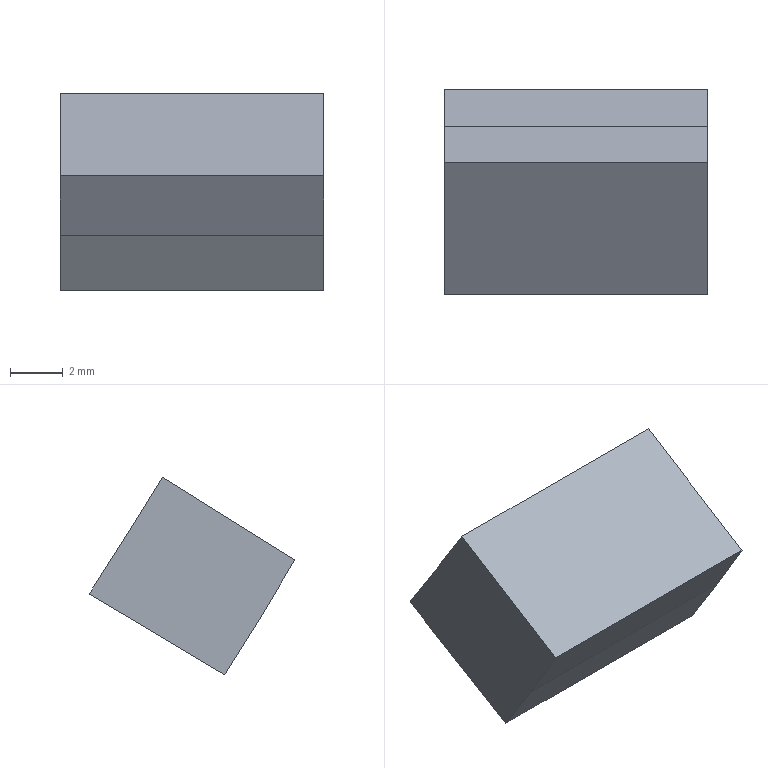Component | SolidWorks | Key5x5x16-2 | 1 solid | 8 faces | box 10 x 7.8 x 7.49 mm | volume 308 mm3 | plane 8
build123d program:
from build123d import *

# Parameters (mm, degrees)
BOSS_EXTRUDE1_DEPTH = 10


with BuildPart() as part:
    # Sketch1 → Boss-Extrude1 (new body)
    with BuildSketch(Plane.XY):
        Polygon((5.447, 152.957), (2.855, 152.957), (2.855, 147.043), (5.474, 146.989), (7.957, 146.989), (8.084, 152.969), align=None)
    extrude(amount=BOSS_EXTRUDE1_DEPTH)


solid = part.part

# Placed as in the assembly
solid = solid.moved(Location((133.654, 14.855, -81.716), (31.981, 90, 0)))
STEP:
#1=COLOUR_RGB('',0.7922,0.8196,0.9333);
#2=FILL_AREA_STYLE_COLOUR('',#1);
#3=FILL_AREA_STYLE('',(#2));
#4=SURFACE_STYLE_FILL_AREA(#3);
#5=SURFACE_SIDE_STYLE('',(#4));
#6=SURFACE_STYLE_USAGE(.BOTH.,#5);
#7=PRESENTATION_STYLE_ASSIGNMENT((#6));
#8=CARTESIAN_POINT('',(5.262,5.862,-0.2975));
#9=VERTEX_POINT('',#8);
#10=CARTESIAN_POINT('',(5.262,5.806,-0.2097));
#11=VERTEX_POINT('',#10);
#12=CARTESIAN_POINT('',(5.262,5.862,-0.2975));
#13=DIRECTION('',(0.,-0.5334,0.8458));
#14=VECTOR('',#13,39.37);
#15=LINE('',#12,#14);
#16=EDGE_CURVE('',#9,#11,#15,.T.);
#17=ORIENTED_EDGE('',*,*,#16,.T.);
#18=CARTESIAN_POINT('',(5.656,5.806,-0.2097));
#19=VERTEX_POINT('',#18);
#20=CARTESIAN_POINT('',(5.656,5.806,-0.2097));
#21=DIRECTION('',(-1.,0.,0.));
#22=VECTOR('',#21,39.37);
#23=LINE('',#20,#22);
#24=EDGE_CURVE('',#19,#11,#23,.T.);
#25=ORIENTED_EDGE('',*,*,#24,.F.);
#26=CARTESIAN_POINT('',(5.656,5.862,-0.2975));
#27=VERTEX_POINT('',#26);
#28=CARTESIAN_POINT('',(5.656,5.862,-0.2975));
#29=DIRECTION('',(0.,-0.5334,0.8458));
#30=VECTOR('',#29,39.37);
#31=LINE('',#28,#30);
#32=EDGE_CURVE('',#27,#19,#31,.T.);
#33=ORIENTED_EDGE('',*,*,#32,.F.);
#34=CARTESIAN_POINT('',(5.656,5.862,-0.2975));
#35=DIRECTION('',(-1.,0.,0.));
#36=VECTOR('',#35,39.37);
#37=LINE('',#34,#36);
#38=EDGE_CURVE('',#27,#9,#37,.T.);
#39=ORIENTED_EDGE('',*,*,#38,.T.);
#40=EDGE_LOOP('',(#17,#25,#33,#39));
#41=FACE_OUTER_BOUND('',#40,.T.);
#42=CARTESIAN_POINT('',(5.656,5.862,-0.2975));
#43=DIRECTION('',(-0.,-0.8458,-0.5334));
#44=DIRECTION('',(-0.,0.5334,-0.8458));
#45=AXIS2_PLACEMENT_3D('',#42,#43,#44);
#46=PLANE('',#45);
#47=ADVANCED_FACE('',(#41),#46,.F.);
#48=CARTESIAN_POINT('',(5.262,5.752,-0.1231));
#49=VERTEX_POINT('',#48);
#50=CARTESIAN_POINT('',(5.262,5.806,-0.2097));
#51=DIRECTION('',(0.,-0.5296,0.8482));
#52=VECTOR('',#51,39.37);
#53=LINE('',#50,#52);
#54=EDGE_CURVE('',#11,#49,#53,.T.);
#55=ORIENTED_EDGE('',*,*,#54,.T.);
#56=CARTESIAN_POINT('',(5.656,5.752,-0.1231));
#57=VERTEX_POINT('',#56);
#58=CARTESIAN_POINT('',(5.656,5.752,-0.1231));
#59=DIRECTION('',(-1.,0.,0.));
#60=VECTOR('',#59,39.37);
#61=LINE('',#58,#60);
#62=EDGE_CURVE('',#57,#49,#61,.T.);
#63=ORIENTED_EDGE('',*,*,#62,.F.);
#64=CARTESIAN_POINT('',(5.656,5.806,-0.2097));
#65=DIRECTION('',(0.,-0.5296,0.8482));
#66=VECTOR('',#65,39.37);
#67=LINE('',#64,#66);
#68=EDGE_CURVE('',#19,#57,#67,.T.);
#69=ORIENTED_EDGE('',*,*,#68,.F.);
#70=ORIENTED_EDGE('',*,*,#24,.T.);
#71=EDGE_LOOP('',(#55,#63,#69,#70));
#72=FACE_OUTER_BOUND('',#71,.T.);
#73=CARTESIAN_POINT('',(5.656,5.806,-0.2097));
#74=DIRECTION('',(-0.,-0.8482,-0.5296));
#75=DIRECTION('',(-1.,0.,0.));
#76=AXIS2_PLACEMENT_3D('',#73,#74,#75);
#77=PLANE('',#76);
#78=ADVANCED_FACE('',(#72),#77,.F.);
#79=CARTESIAN_POINT('',(5.262,5.555,-0.2464));
#80=VERTEX_POINT('',#79);
#81=CARTESIAN_POINT('',(5.262,5.752,-0.1231));
#82=DIRECTION('',(-0.,-0.8482,-0.5296));
#83=VECTOR('',#82,39.37);
#84=LINE('',#81,#83);
#85=EDGE_CURVE('',#49,#80,#84,.T.);
#86=ORIENTED_EDGE('',*,*,#85,.T.);
#87=CARTESIAN_POINT('',(5.656,5.555,-0.2464));
#88=VERTEX_POINT('',#87);
#89=CARTESIAN_POINT('',(5.656,5.555,-0.2464));
#90=DIRECTION('',(-1.,0.,0.));
#91=VECTOR('',#90,39.37);
#92=LINE('',#89,#91);
#93=EDGE_CURVE('',#88,#80,#92,.T.);
#94=ORIENTED_EDGE('',*,*,#93,.F.);
#95=CARTESIAN_POINT('',(5.656,5.752,-0.1231));
#96=DIRECTION('',(-0.,-0.8482,-0.5296));
#97=VECTOR('',#96,39.37);
#98=LINE('',#95,#97);
#99=EDGE_CURVE('',#57,#88,#98,.T.);
#100=ORIENTED_EDGE('',*,*,#99,.F.);
#101=ORIENTED_EDGE('',*,*,#62,.T.);
#102=EDGE_LOOP('',(#86,#94,#100,#101));
#103=FACE_OUTER_BOUND('',#102,.T.);
#104=CARTESIAN_POINT('',(5.656,5.752,-0.1231));
#105=DIRECTION('',(-0.,0.5296,-0.8482));
#106=DIRECTION('',(-1.,0.,0.));
#107=AXIS2_PLACEMENT_3D('',#104,#105,#106);
#108=PLANE('',#107);
#109=ADVANCED_FACE('',(#103),#108,.F.);
#110=CARTESIAN_POINT('',(5.262,5.608,-0.335));
#111=VERTEX_POINT('',#110);
#112=CARTESIAN_POINT('',(5.262,5.555,-0.2464));
#113=DIRECTION('',(-0.,0.5121,-0.8589));
#114=VECTOR('',#113,39.37);
#115=LINE('',#112,#114);
#116=EDGE_CURVE('',#80,#111,#115,.T.);
#117=ORIENTED_EDGE('',*,*,#116,.T.);
#118=CARTESIAN_POINT('',(5.656,5.608,-0.335));
#119=VERTEX_POINT('',#118);
#120=CARTESIAN_POINT('',(5.656,5.608,-0.335));
#121=DIRECTION('',(-1.,0.,0.));
#122=VECTOR('',#121,39.37);
#123=LINE('',#120,#122);
#124=EDGE_CURVE('',#119,#111,#123,.T.);
#125=ORIENTED_EDGE('',*,*,#124,.F.);
#126=CARTESIAN_POINT('',(5.656,5.555,-0.2464));
#127=DIRECTION('',(-0.,0.5121,-0.8589));
#128=VECTOR('',#127,39.37);
#129=LINE('',#126,#128);
#130=EDGE_CURVE('',#88,#119,#129,.T.);
#131=ORIENTED_EDGE('',*,*,#130,.F.);
#132=ORIENTED_EDGE('',*,*,#93,.T.);
#133=EDGE_LOOP('',(#117,#125,#131,#132));
#134=FACE_OUTER_BOUND('',#133,.T.);
#135=CARTESIAN_POINT('',(5.656,5.555,-0.2464));
#136=DIRECTION('',(0.,0.8589,0.5121));
#137=DIRECTION('',(0.,-0.5121,0.8589));
#138=AXIS2_PLACEMENT_3D('',#135,#136,#137);
#139=PLANE('',#138);
#140=ADVANCED_FACE('',(#134),#139,.F.);
#141=CARTESIAN_POINT('',(5.262,5.659,-0.4179));
#142=VERTEX_POINT('',#141);
#143=CARTESIAN_POINT('',(5.262,5.608,-0.335));
#144=DIRECTION('',(-0.,0.5296,-0.8482));
#145=VECTOR('',#144,39.37);
#146=LINE('',#143,#145);
#147=EDGE_CURVE('',#111,#142,#146,.T.);
#148=ORIENTED_EDGE('',*,*,#147,.T.);
#149=CARTESIAN_POINT('',(5.656,5.659,-0.4179));
#150=VERTEX_POINT('',#149);
#151=CARTESIAN_POINT('',(5.656,5.659,-0.4179));
#152=DIRECTION('',(-1.,0.,0.));
#153=VECTOR('',#152,39.37);
#154=LINE('',#151,#153);
#155=EDGE_CURVE('',#150,#142,#154,.T.);
#156=ORIENTED_EDGE('',*,*,#155,.F.);
#157=CARTESIAN_POINT('',(5.656,5.608,-0.335));
#158=DIRECTION('',(-0.,0.5296,-0.8482));
#159=VECTOR('',#158,39.37);
#160=LINE('',#157,#159);
#161=EDGE_CURVE('',#119,#150,#160,.T.);
#162=ORIENTED_EDGE('',*,*,#161,.F.);
#163=ORIENTED_EDGE('',*,*,#124,.T.);
#164=EDGE_LOOP('',(#148,#156,#162,#163));
#165=FACE_OUTER_BOUND('',#164,.T.);
#166=CARTESIAN_POINT('',(5.656,5.608,-0.335));
#167=DIRECTION('',(0.,0.8482,0.5296));
#168=DIRECTION('',(1.,-0.,-0.));
#169=AXIS2_PLACEMENT_3D('',#166,#167,#168);
#170=PLANE('',#169);
#171=ADVANCED_FACE('',(#165),#170,.F.);
#172=CARTESIAN_POINT('',(5.262,5.862,-0.2975));
#173=DIRECTION('',(0.,0.8593,0.5115));
#174=VECTOR('',#173,39.37);
#175=LINE('',#172,#174);
#176=EDGE_CURVE('',#142,#9,#175,.T.);
#177=ORIENTED_EDGE('',*,*,#176,.T.);
#178=ORIENTED_EDGE('',*,*,#38,.F.);
#179=CARTESIAN_POINT('',(5.656,5.862,-0.2975));
#180=DIRECTION('',(0.,0.8593,0.5115));
#181=VECTOR('',#180,39.37);
#182=LINE('',#179,#181);
#183=EDGE_CURVE('',#150,#27,#182,.T.);
#184=ORIENTED_EDGE('',*,*,#183,.F.);
#185=ORIENTED_EDGE('',*,*,#155,.T.);
#186=EDGE_LOOP('',(#177,#178,#184,#185));
#187=FACE_OUTER_BOUND('',#186,.T.);
#188=CARTESIAN_POINT('',(5.656,5.862,-0.2975));
#189=DIRECTION('',(0.,-0.5115,0.8593));
#190=DIRECTION('',(-0.,-0.8593,-0.5115));
#191=AXIS2_PLACEMENT_3D('',#188,#189,#190);
#192=PLANE('',#191);
#193=ADVANCED_FACE('',(#187),#192,.F.);
#194=ORIENTED_EDGE('',*,*,#32,.T.);
#195=ORIENTED_EDGE('',*,*,#68,.T.);
#196=ORIENTED_EDGE('',*,*,#99,.T.);
#197=ORIENTED_EDGE('',*,*,#130,.T.);
#198=ORIENTED_EDGE('',*,*,#161,.T.);
#199=ORIENTED_EDGE('',*,*,#183,.T.);
#200=EDGE_LOOP('',(#194,#195,#196,#197,#198,#199));
#201=FACE_OUTER_BOUND('',#200,.T.);
#202=CARTESIAN_POINT('',(5.656,0.5848,-3.217));
#203=DIRECTION('',(1.,-0.,-0.));
#204=DIRECTION('',(-0.,0.5296,-0.8482));
#205=AXIS2_PLACEMENT_3D('',#202,#203,#204);
#206=PLANE('',#205);
#207=ADVANCED_FACE('',(#201),#206,.T.);
#208=ORIENTED_EDGE('',*,*,#16,.F.);
#209=ORIENTED_EDGE('',*,*,#176,.F.);
#210=ORIENTED_EDGE('',*,*,#147,.F.);
#211=ORIENTED_EDGE('',*,*,#116,.F.);
#212=ORIENTED_EDGE('',*,*,#85,.F.);
#213=ORIENTED_EDGE('',*,*,#54,.F.);
#214=EDGE_LOOP('',(#208,#209,#210,#211,#212,#213));
#215=FACE_OUTER_BOUND('',#214,.T.);
#216=CARTESIAN_POINT('',(5.262,0.5848,-3.217));
#217=DIRECTION('',(1.,-0.,-0.));
#218=DIRECTION('',(-0.,0.5296,-0.8482));
#219=AXIS2_PLACEMENT_3D('',#216,#217,#218);
#220=PLANE('',#219);
#221=ADVANCED_FACE('',(#215),#220,.F.);
#222=CLOSED_SHELL('',(#47,#78,#109,#140,#171,#193,#207,#221));
#223=MANIFOLD_SOLID_BREP('',#222);
#224=STYLED_ITEM('',(#7),#223);
#225=(LENGTH_UNIT()NAMED_UNIT(*)SI_UNIT($,.METRE.));
#226=LENGTH_MEASURE_WITH_UNIT(LENGTH_MEASURE(0.0254),#225);
#227=DIMENSIONAL_EXPONENTS(1.,0.,0.,0.,0.,0.,0.);
#228=(CONVERSION_BASED_UNIT('',#226)LENGTH_UNIT()NAMED_UNIT(#227));
#229=UNCERTAINTY_MEASURE_WITH_UNIT(LENGTH_MEASURE(0.00001),#228,'','');
#230=(NAMED_UNIT(*)PLANE_ANGLE_UNIT()SI_UNIT($,.RADIAN.));
#231=(NAMED_UNIT(*)SI_UNIT($,.STERADIAN.)SOLID_ANGLE_UNIT());
#232=(GEOMETRIC_REPRESENTATION_CONTEXT(3)GLOBAL_UNCERTAINTY_ASSIGNED_CONTEXT((#229))GLOBAL_UNIT_ASSIGNED_CONTEXT((#228,#230,#231))REPRESENTATION_CONTEXT('',''));
#233=MECHANICAL_DESIGN_GEOMETRIC_PRESENTATION_REPRESENTATION('',(#224),#232);
#234=PRESENTATION_LAYER_ASSIGNMENT('','',(#224));
#235=CARTESIAN_POINT('',(0.,0.,0.));
#236=DIRECTION('',(0.,0.,1.));
#237=DIRECTION('',(1.,0.,0.));
#238=AXIS2_PLACEMENT_3D('',#235,#236,#237);
#239=(LENGTH_UNIT()NAMED_UNIT(*)SI_UNIT($,.METRE.));
#240=LENGTH_MEASURE_WITH_UNIT(LENGTH_MEASURE(0.0254),#239);
#241=DIMENSIONAL_EXPONENTS(1.,0.,0.,0.,0.,0.,0.);
#242=(CONVERSION_BASED_UNIT('',#240)LENGTH_UNIT()NAMED_UNIT(#241));
#243=UNCERTAINTY_MEASURE_WITH_UNIT(LENGTH_MEASURE(0.00001),#242,'','');
#244=(NAMED_UNIT(*)PLANE_ANGLE_UNIT()SI_UNIT($,.RADIAN.));
#245=(NAMED_UNIT(*)SI_UNIT($,.STERADIAN.)SOLID_ANGLE_UNIT());
#246=(GEOMETRIC_REPRESENTATION_CONTEXT(3)GLOBAL_UNCERTAINTY_ASSIGNED_CONTEXT((#243))GLOBAL_UNIT_ASSIGNED_CONTEXT((#242,#244,#245))REPRESENTATION_CONTEXT('',''));
#247=ADVANCED_BREP_SHAPE_REPRESENTATION('',(#223,#238),#246);